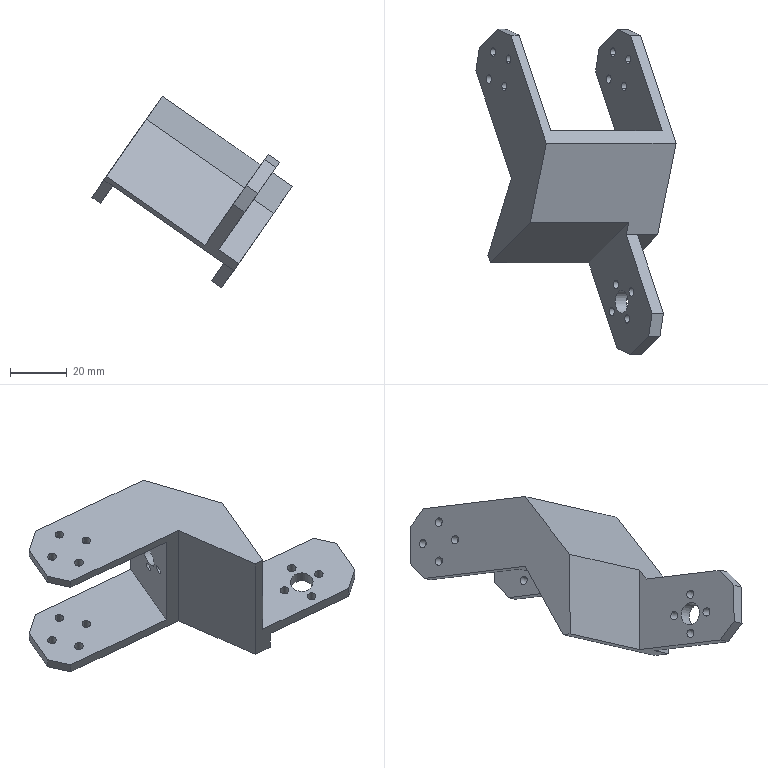Component | NX | U_SHAPE_3 | 1 solid | 53 faces | volume 51474 mm3 | plane 29 | other 17 | cylinder 7 | commonest cylinder face diameters 3 x6 8 x1